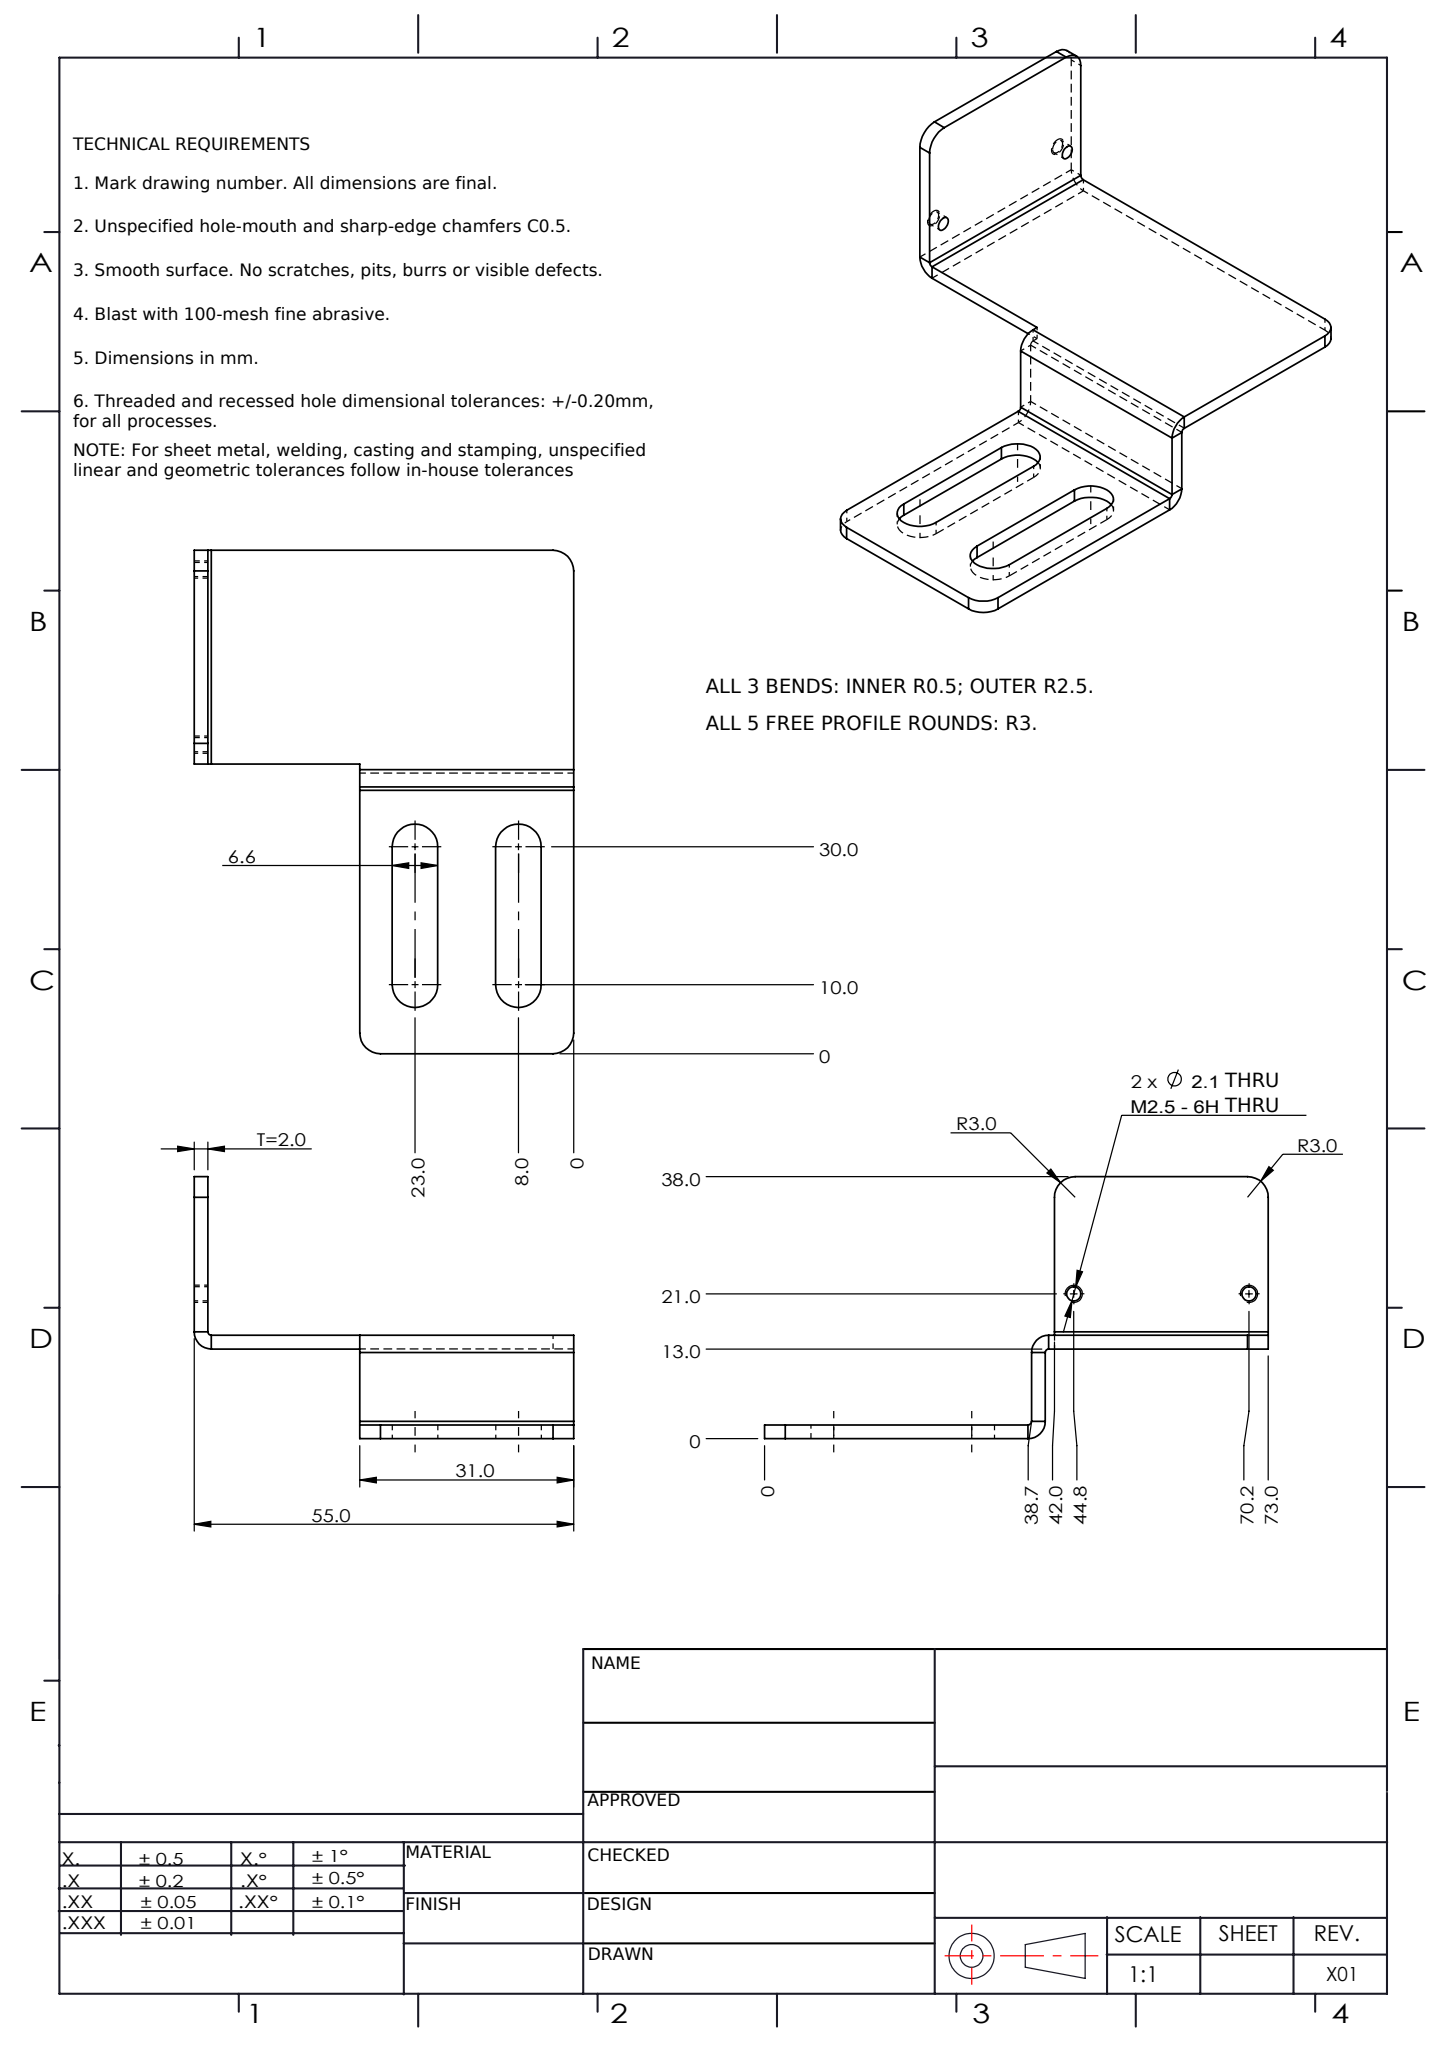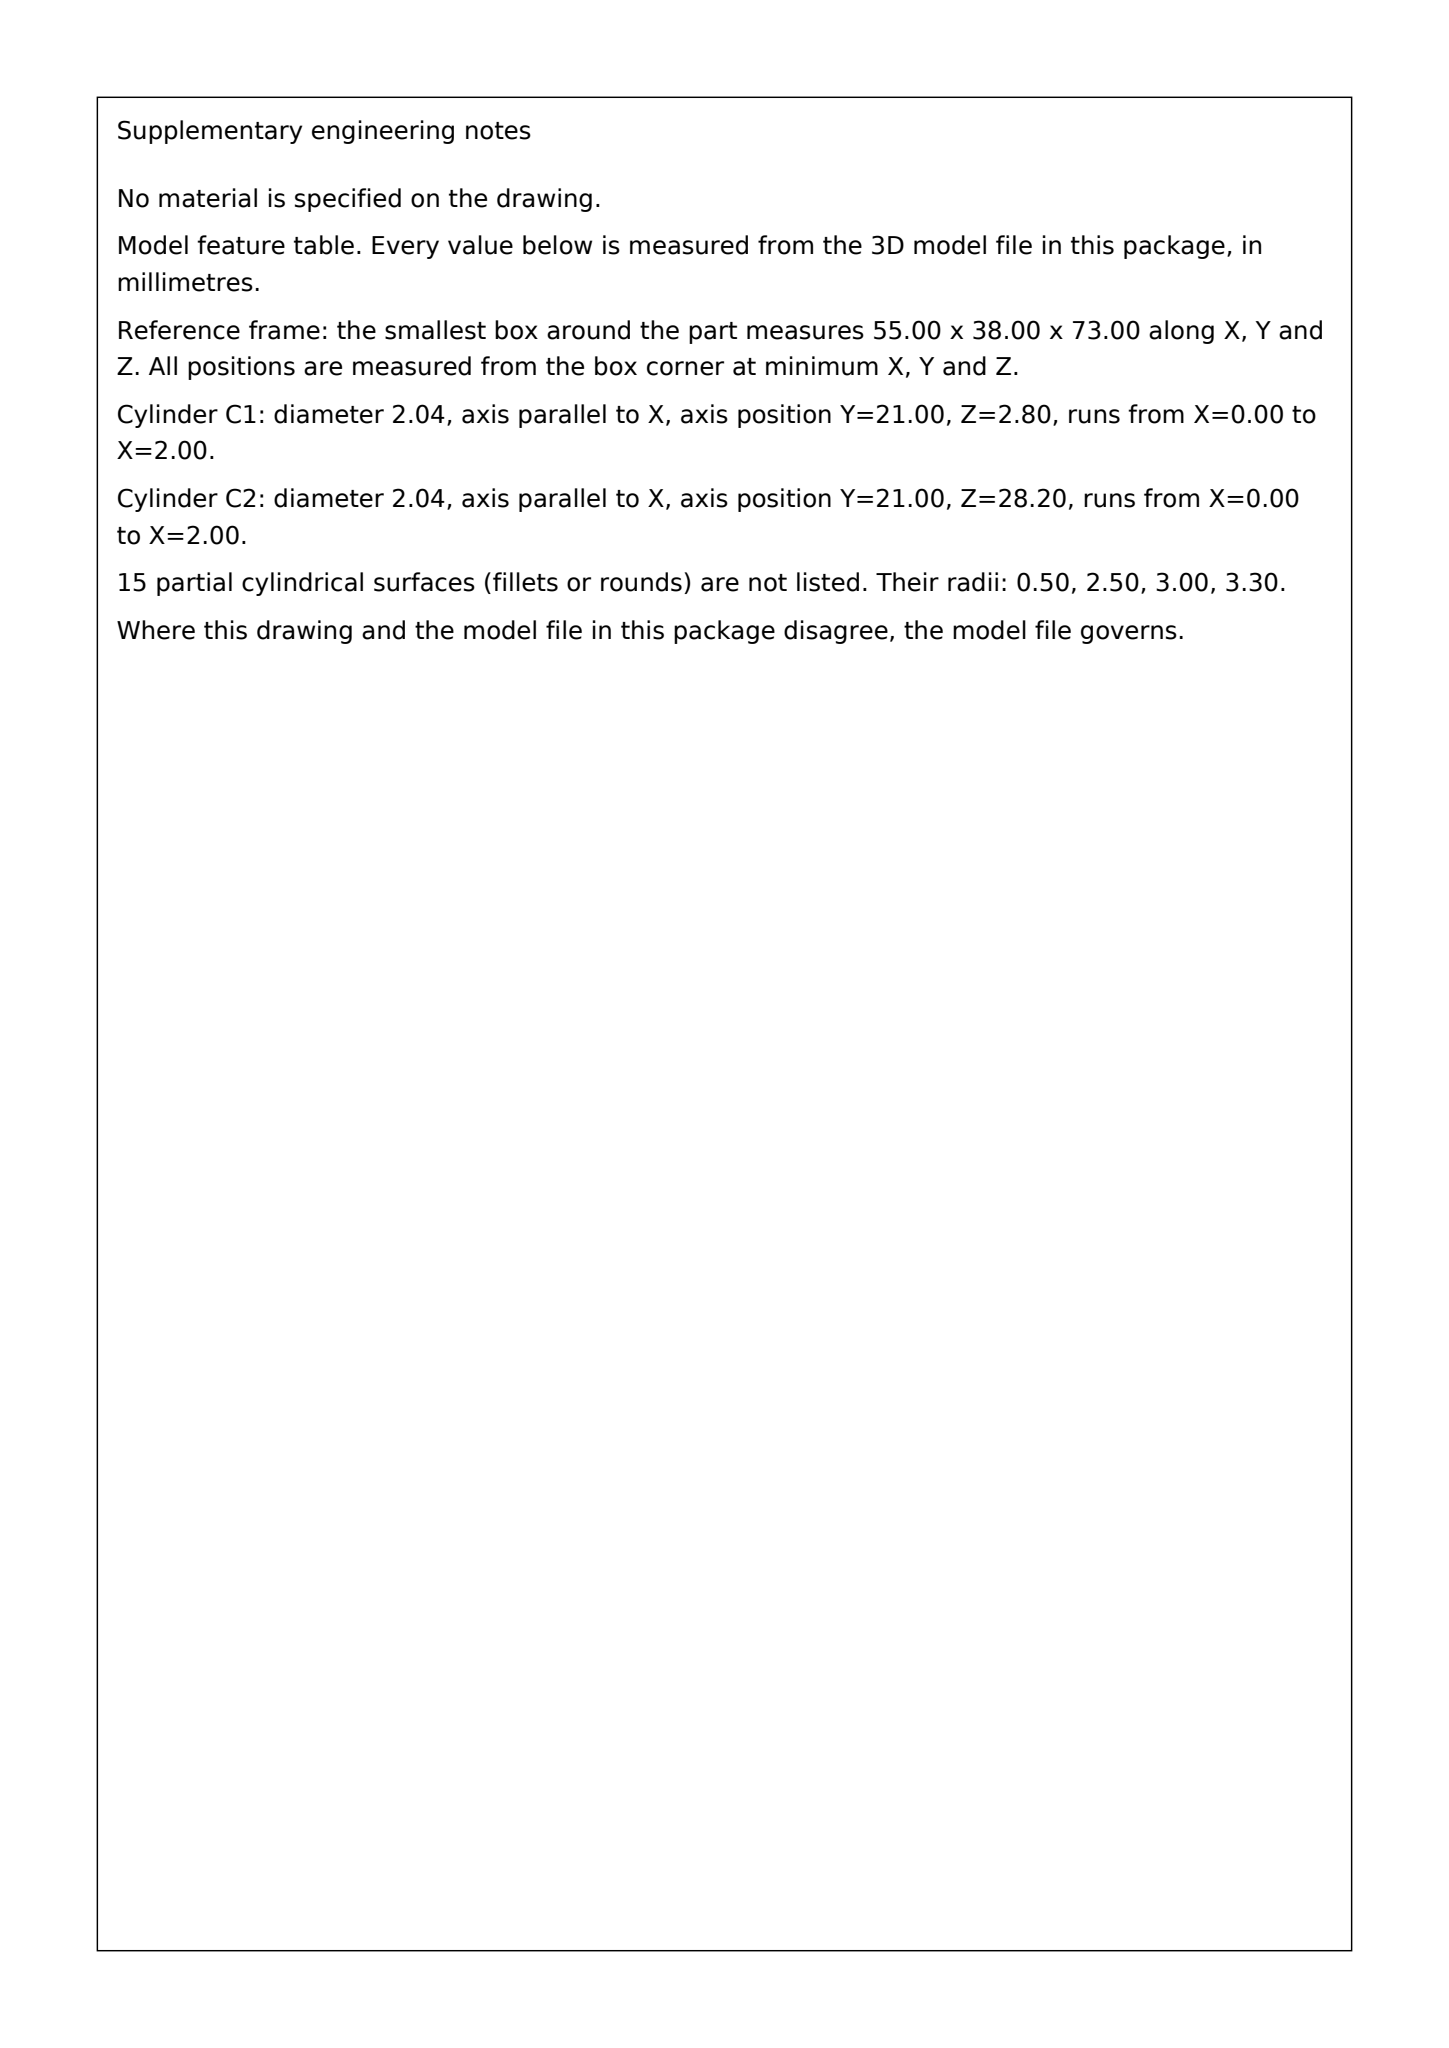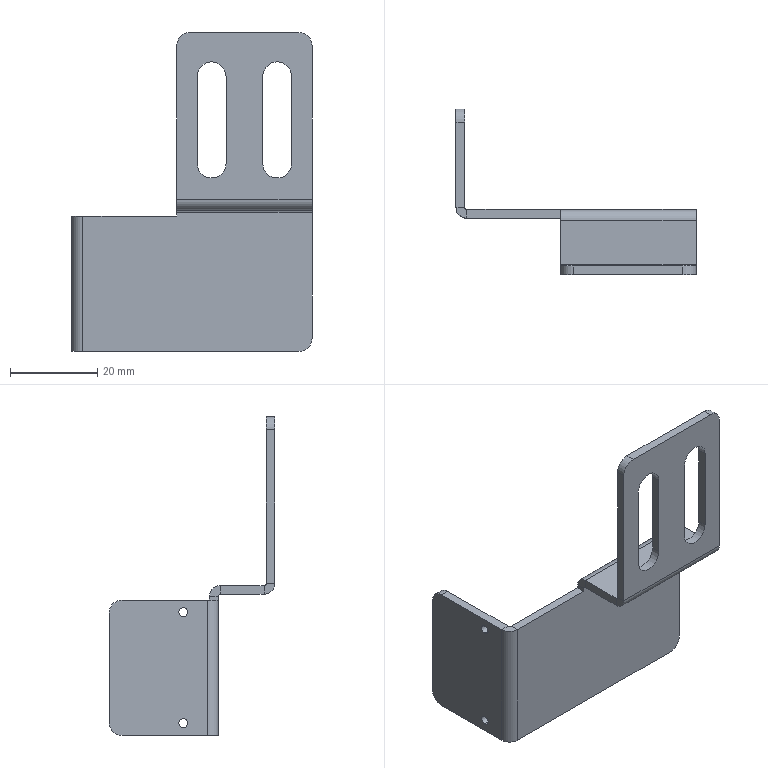Part | SolidWorks | mm | 1 solid | 51 faces | box 55 x 38 x 73 mm | volume 7429 mm3 | plane 30 | cylinder 21 | commonest cylinder face diameters 6.6 x6 6 x5 2.05 x4 1 x3 5 x3